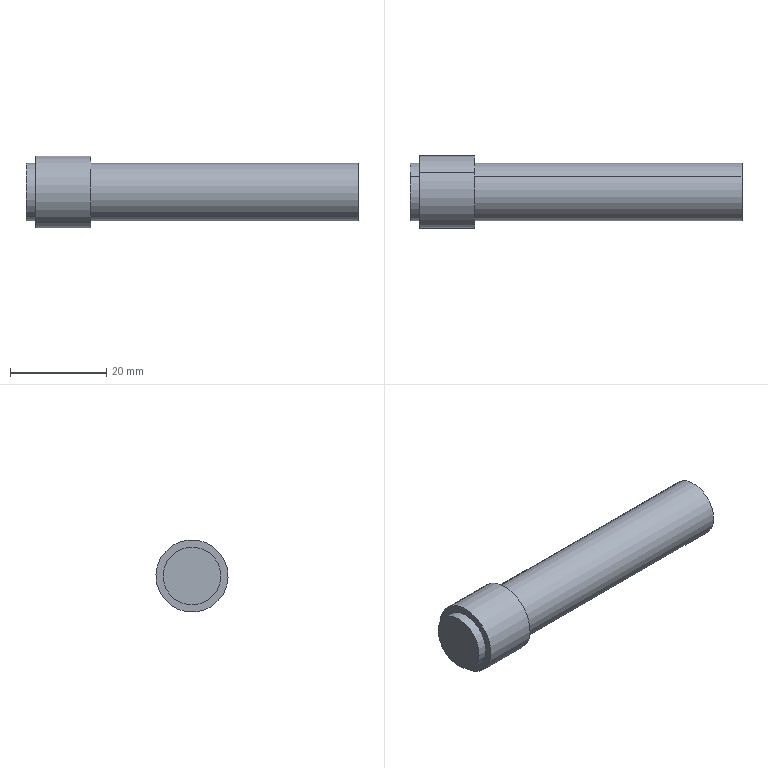Component | SolidWorks | GearShaft-4 | 1 solid | 10 faces | box 69 x 15 x 15 mm | volume 8535 mm3 | cylinder 6 | plane 4 | commonest cylinder face diameters 12 x4 15 x2
build123d program:
from build123d import *

# Parameters (mm, degrees)
BOSS_EXTRUDE1_DEPTH      = 14
BOSS_EXTRUDE1_DEPTH_BACK = 55
SKETCH1_R                = 6
BOSS_EXTRUDE2_START      = -2
SKETCH2_R                = 7.5
BOSS_EXTRUDE2_DEPTH      = 11.5


with BuildPart() as part:
    # Sketch1 → Boss-Extrude1 (new, two sides: drawn at the far end of the back side and taken through both)
    with BuildSketch(Plane.XY.offset(-BOSS_EXTRUDE1_DEPTH_BACK)):
        with Locations((-64.2, 0)):
            Circle(SKETCH1_R)
    extrude(amount=BOSS_EXTRUDE1_DEPTH + BOSS_EXTRUDE1_DEPTH_BACK)

    # Sketch2 → Boss-Extrude2 (add)
    with BuildSketch(Plane.XY.offset(14).offset(BOSS_EXTRUDE2_START)):
        with Locations((-64.2, 0)):
            Circle(SKETCH2_R)
    extrude(amount=-BOSS_EXTRUDE2_DEPTH)


solid = part.part

# Placed as in the assembly
solid = solid.moved(Location((-42.875, -67.172, 107.182), (0, -90, 0)))
STEP:
#1=COLOUR_RGB('',0.7922,0.8196,0.9333);
#2=FILL_AREA_STYLE_COLOUR('',#1);
#3=FILL_AREA_STYLE('',(#2));
#4=SURFACE_STYLE_FILL_AREA(#3);
#5=SURFACE_SIDE_STYLE('',(#4));
#6=SURFACE_STYLE_USAGE(.BOTH.,#5);
#7=PRESENTATION_STYLE_ASSIGNMENT((#6));
#8=CARTESIAN_POINT('',(-2.16,-2.518,1.892));
#9=VERTEX_POINT('',#8);
#10=CARTESIAN_POINT('',(-2.16,-2.771,1.493));
#11=VERTEX_POINT('',#10);
#12=CARTESIAN_POINT('',(-2.16,-2.645,1.692));
#13=DIRECTION('',(1.,0.,0.));
#14=DIRECTION('',(0.,-0.5345,-0.8452));
#15=AXIS2_PLACEMENT_3D('',#12,#13,#14);
#16=CIRCLE('',#15,0.2362);
#17=EDGE_CURVE('',#9,#11,#16,.T.);
#18=ORIENTED_EDGE('',*,*,#17,.F.);
#19=CARTESIAN_POINT('',(-2.239,-2.518,1.892));
#20=VERTEX_POINT('',#19);
#21=CARTESIAN_POINT('',(0.4773,-2.518,1.892));
#22=DIRECTION('',(-1.,-0.,-0.));
#23=VECTOR('',#22,39.37);
#24=LINE('',#21,#23);
#25=EDGE_CURVE('',#9,#20,#24,.T.);
#26=ORIENTED_EDGE('',*,*,#25,.T.);
#27=CARTESIAN_POINT('',(-2.239,-2.771,1.493));
#28=VERTEX_POINT('',#27);
#29=CARTESIAN_POINT('',(-2.239,-2.645,1.692));
#30=DIRECTION('',(-1.,-0.,-0.));
#31=DIRECTION('',(0.,-0.5345,-0.8452));
#32=AXIS2_PLACEMENT_3D('',#29,#30,#31);
#33=CIRCLE('',#32,0.2362);
#34=EDGE_CURVE('',#28,#20,#33,.T.);
#35=ORIENTED_EDGE('',*,*,#34,.F.);
#36=CARTESIAN_POINT('',(0.4773,-2.771,1.493));
#37=DIRECTION('',(-1.,-0.,-0.));
#38=VECTOR('',#37,39.37);
#39=LINE('',#36,#38);
#40=EDGE_CURVE('',#11,#28,#39,.T.);
#41=ORIENTED_EDGE('',*,*,#40,.F.);
#42=EDGE_LOOP('',(#18,#26,#35,#41));
#43=FACE_OUTER_BOUND('',#42,.T.);
#44=CARTESIAN_POINT('',(0.4773,-2.645,1.692));
#45=DIRECTION('',(-1.,-0.,-0.));
#46=DIRECTION('',(0.,-0.5345,-0.8452));
#47=AXIS2_PLACEMENT_3D('',#44,#45,#46);
#48=CYLINDRICAL_SURFACE('',#47,0.2362);
#49=ADVANCED_FACE('',(#43),#48,.T.);
#50=CARTESIAN_POINT('',(-1.708,-2.802,1.443));
#51=VERTEX_POINT('',#50);
#52=CARTESIAN_POINT('',(-1.708,-2.487,1.942));
#53=VERTEX_POINT('',#52);
#54=CARTESIAN_POINT('',(-1.708,-2.645,1.692));
#55=DIRECTION('',(-1.,-0.,-0.));
#56=DIRECTION('',(0.,-0.5345,-0.8452));
#57=AXIS2_PLACEMENT_3D('',#54,#55,#56);
#58=CIRCLE('',#57,0.2953);
#59=EDGE_CURVE('',#51,#53,#58,.T.);
#60=ORIENTED_EDGE('',*,*,#59,.T.);
#61=CARTESIAN_POINT('',(-2.16,-2.487,1.942));
#62=VERTEX_POINT('',#61);
#63=CARTESIAN_POINT('',(-1.708,-2.487,1.942));
#64=DIRECTION('',(-1.,-0.,-0.));
#65=VECTOR('',#64,39.37);
#66=LINE('',#63,#65);
#67=EDGE_CURVE('',#53,#62,#66,.T.);
#68=ORIENTED_EDGE('',*,*,#67,.T.);
#69=CARTESIAN_POINT('',(-2.16,-2.802,1.443));
#70=VERTEX_POINT('',#69);
#71=CARTESIAN_POINT('',(-2.16,-2.645,1.692));
#72=DIRECTION('',(-1.,-0.,-0.));
#73=DIRECTION('',(0.,-0.5345,-0.8452));
#74=AXIS2_PLACEMENT_3D('',#71,#72,#73);
#75=CIRCLE('',#74,0.2953);
#76=EDGE_CURVE('',#70,#62,#75,.T.);
#77=ORIENTED_EDGE('',*,*,#76,.F.);
#78=CARTESIAN_POINT('',(-1.708,-2.802,1.443));
#79=DIRECTION('',(-1.,-0.,-0.));
#80=VECTOR('',#79,39.37);
#81=LINE('',#78,#80);
#82=EDGE_CURVE('',#51,#70,#81,.T.);
#83=ORIENTED_EDGE('',*,*,#82,.F.);
#84=EDGE_LOOP('',(#60,#68,#77,#83));
#85=FACE_OUTER_BOUND('',#84,.T.);
#86=CARTESIAN_POINT('',(-1.708,-2.645,1.692));
#87=DIRECTION('',(-1.,-0.,-0.));
#88=DIRECTION('',(0.,-0.5345,-0.8452));
#89=AXIS2_PLACEMENT_3D('',#86,#87,#88);
#90=CYLINDRICAL_SURFACE('',#89,0.2953);
#91=ADVANCED_FACE('',(#85),#90,.T.);
#92=CARTESIAN_POINT('',(0.4773,-2.771,1.493));
#93=VERTEX_POINT('',#92);
#94=CARTESIAN_POINT('',(0.4773,-2.518,1.892));
#95=VERTEX_POINT('',#94);
#96=CARTESIAN_POINT('',(0.4773,-2.645,1.692));
#97=DIRECTION('',(-1.,-0.,-0.));
#98=DIRECTION('',(0.,-0.5345,-0.8452));
#99=AXIS2_PLACEMENT_3D('',#96,#97,#98);
#100=CIRCLE('',#99,0.2362);
#101=EDGE_CURVE('',#93,#95,#100,.T.);
#102=ORIENTED_EDGE('',*,*,#101,.T.);
#103=CARTESIAN_POINT('',(-1.708,-2.518,1.892));
#104=VERTEX_POINT('',#103);
#105=CARTESIAN_POINT('',(0.4773,-2.518,1.892));
#106=DIRECTION('',(-1.,-0.,-0.));
#107=VECTOR('',#106,39.37);
#108=LINE('',#105,#107);
#109=EDGE_CURVE('',#95,#104,#108,.T.);
#110=ORIENTED_EDGE('',*,*,#109,.T.);
#111=CARTESIAN_POINT('',(-1.708,-2.771,1.493));
#112=VERTEX_POINT('',#111);
#113=CARTESIAN_POINT('',(-1.708,-2.645,1.692));
#114=DIRECTION('',(1.,0.,0.));
#115=DIRECTION('',(0.,-0.5345,-0.8452));
#116=AXIS2_PLACEMENT_3D('',#113,#114,#115);
#117=CIRCLE('',#116,0.2362);
#118=EDGE_CURVE('',#104,#112,#117,.T.);
#119=ORIENTED_EDGE('',*,*,#118,.T.);
#120=CARTESIAN_POINT('',(0.4773,-2.771,1.493));
#121=DIRECTION('',(-1.,-0.,-0.));
#122=VECTOR('',#121,39.37);
#123=LINE('',#120,#122);
#124=EDGE_CURVE('',#93,#112,#123,.T.);
#125=ORIENTED_EDGE('',*,*,#124,.F.);
#126=EDGE_LOOP('',(#102,#110,#119,#125));
#127=FACE_OUTER_BOUND('',#126,.T.);
#128=CARTESIAN_POINT('',(0.4773,-2.645,1.692));
#129=DIRECTION('',(-1.,-0.,-0.));
#130=DIRECTION('',(0.,-0.5345,-0.8452));
#131=AXIS2_PLACEMENT_3D('',#128,#129,#130);
#132=CYLINDRICAL_SURFACE('',#131,0.2362);
#133=ADVANCED_FACE('',(#127),#132,.T.);
#134=ORIENTED_EDGE('',*,*,#109,.F.);
#135=CARTESIAN_POINT('',(0.4773,-2.645,1.692));
#136=DIRECTION('',(-1.,-0.,-0.));
#137=DIRECTION('',(0.,-0.5345,-0.8452));
#138=AXIS2_PLACEMENT_3D('',#135,#136,#137);
#139=CIRCLE('',#138,0.2362);
#140=EDGE_CURVE('',#95,#93,#139,.T.);
#141=ORIENTED_EDGE('',*,*,#140,.T.);
#142=ORIENTED_EDGE('',*,*,#124,.T.);
#143=CARTESIAN_POINT('',(-1.708,-2.645,1.692));
#144=DIRECTION('',(1.,0.,0.));
#145=DIRECTION('',(0.,-0.5345,-0.8452));
#146=AXIS2_PLACEMENT_3D('',#143,#144,#145);
#147=CIRCLE('',#146,0.2362);
#148=EDGE_CURVE('',#112,#104,#147,.T.);
#149=ORIENTED_EDGE('',*,*,#148,.T.);
#150=EDGE_LOOP('',(#134,#141,#142,#149));
#151=FACE_OUTER_BOUND('',#150,.T.);
#152=CARTESIAN_POINT('',(0.4773,-2.645,1.692));
#153=DIRECTION('',(-1.,-0.,-0.));
#154=DIRECTION('',(0.,-0.5345,-0.8452));
#155=AXIS2_PLACEMENT_3D('',#152,#153,#154);
#156=CYLINDRICAL_SURFACE('',#155,0.2362);
#157=ADVANCED_FACE('',(#151),#156,.T.);
#158=ORIENTED_EDGE('',*,*,#101,.F.);
#159=ORIENTED_EDGE('',*,*,#140,.F.);
#160=EDGE_LOOP('',(#158,#159));
#161=FACE_OUTER_BOUND('',#160,.T.);
#162=CARTESIAN_POINT('',(0.4773,-2.645,1.692));
#163=DIRECTION('',(-1.,-0.,-0.));
#164=DIRECTION('',(0.,-0.5345,-0.8452));
#165=AXIS2_PLACEMENT_3D('',#162,#163,#164);
#166=PLANE('',#165);
#167=ADVANCED_FACE('',(#161),#166,.F.);
#168=ORIENTED_EDGE('',*,*,#67,.F.);
#169=CARTESIAN_POINT('',(-1.708,-2.645,1.692));
#170=DIRECTION('',(-1.,-0.,-0.));
#171=DIRECTION('',(0.,-0.5345,-0.8452));
#172=AXIS2_PLACEMENT_3D('',#169,#170,#171);
#173=CIRCLE('',#172,0.2953);
#174=EDGE_CURVE('',#53,#51,#173,.T.);
#175=ORIENTED_EDGE('',*,*,#174,.T.);
#176=ORIENTED_EDGE('',*,*,#82,.T.);
#177=CARTESIAN_POINT('',(-2.16,-2.645,1.692));
#178=DIRECTION('',(-1.,-0.,-0.));
#179=DIRECTION('',(0.,-0.5345,-0.8452));
#180=AXIS2_PLACEMENT_3D('',#177,#178,#179);
#181=CIRCLE('',#180,0.2953);
#182=EDGE_CURVE('',#62,#70,#181,.T.);
#183=ORIENTED_EDGE('',*,*,#182,.F.);
#184=EDGE_LOOP('',(#168,#175,#176,#183));
#185=FACE_OUTER_BOUND('',#184,.T.);
#186=CARTESIAN_POINT('',(-1.708,-2.645,1.692));
#187=DIRECTION('',(-1.,-0.,-0.));
#188=DIRECTION('',(0.,-0.5345,-0.8452));
#189=AXIS2_PLACEMENT_3D('',#186,#187,#188);
#190=CYLINDRICAL_SURFACE('',#189,0.2953);
#191=ADVANCED_FACE('',(#185),#190,.T.);
#192=ORIENTED_EDGE('',*,*,#148,.F.);
#193=ORIENTED_EDGE('',*,*,#118,.F.);
#194=EDGE_LOOP('',(#192,#193));
#195=FACE_BOUND('',#194,.T.);
#196=ORIENTED_EDGE('',*,*,#59,.F.);
#197=ORIENTED_EDGE('',*,*,#174,.F.);
#198=EDGE_LOOP('',(#196,#197));
#199=FACE_OUTER_BOUND('',#198,.T.);
#200=CARTESIAN_POINT('',(-1.708,-2.645,1.692));
#201=DIRECTION('',(-1.,-0.,-0.));
#202=DIRECTION('',(0.,-0.5345,-0.8452));
#203=AXIS2_PLACEMENT_3D('',#200,#201,#202);
#204=PLANE('',#203);
#205=ADVANCED_FACE('',(#195,#199),#204,.F.);
#206=CARTESIAN_POINT('',(-2.16,-2.645,1.692));
#207=DIRECTION('',(1.,0.,0.));
#208=DIRECTION('',(0.,-0.5345,-0.8452));
#209=AXIS2_PLACEMENT_3D('',#206,#207,#208);
#210=CIRCLE('',#209,0.2362);
#211=EDGE_CURVE('',#11,#9,#210,.T.);
#212=ORIENTED_EDGE('',*,*,#211,.T.);
#213=ORIENTED_EDGE('',*,*,#17,.T.);
#214=EDGE_LOOP('',(#212,#213));
#215=FACE_BOUND('',#214,.T.);
#216=ORIENTED_EDGE('',*,*,#76,.T.);
#217=ORIENTED_EDGE('',*,*,#182,.T.);
#218=EDGE_LOOP('',(#216,#217));
#219=FACE_OUTER_BOUND('',#218,.T.);
#220=CARTESIAN_POINT('',(-2.16,-2.645,1.692));
#221=DIRECTION('',(-1.,-0.,-0.));
#222=DIRECTION('',(0.,-0.5345,-0.8452));
#223=AXIS2_PLACEMENT_3D('',#220,#221,#222);
#224=PLANE('',#223);
#225=ADVANCED_FACE('',(#215,#219),#224,.T.);
#226=ORIENTED_EDGE('',*,*,#34,.T.);
#227=CARTESIAN_POINT('',(-2.239,-2.645,1.692));
#228=DIRECTION('',(-1.,-0.,-0.));
#229=DIRECTION('',(0.,-0.5345,-0.8452));
#230=AXIS2_PLACEMENT_3D('',#227,#228,#229);
#231=CIRCLE('',#230,0.2362);
#232=EDGE_CURVE('',#20,#28,#231,.T.);
#233=ORIENTED_EDGE('',*,*,#232,.T.);
#234=EDGE_LOOP('',(#226,#233));
#235=FACE_OUTER_BOUND('',#234,.T.);
#236=CARTESIAN_POINT('',(-2.239,-2.645,1.692));
#237=DIRECTION('',(-1.,-0.,-0.));
#238=DIRECTION('',(0.,-0.5345,-0.8452));
#239=AXIS2_PLACEMENT_3D('',#236,#237,#238);
#240=PLANE('',#239);
#241=ADVANCED_FACE('',(#235),#240,.T.);
#242=ORIENTED_EDGE('',*,*,#25,.F.);
#243=ORIENTED_EDGE('',*,*,#211,.F.);
#244=ORIENTED_EDGE('',*,*,#40,.T.);
#245=ORIENTED_EDGE('',*,*,#232,.F.);
#246=EDGE_LOOP('',(#242,#243,#244,#245));
#247=FACE_OUTER_BOUND('',#246,.T.);
#248=CARTESIAN_POINT('',(0.4773,-2.645,1.692));
#249=DIRECTION('',(-1.,-0.,-0.));
#250=DIRECTION('',(0.,-0.5345,-0.8452));
#251=AXIS2_PLACEMENT_3D('',#248,#249,#250);
#252=CYLINDRICAL_SURFACE('',#251,0.2362);
#253=ADVANCED_FACE('',(#247),#252,.T.);
#254=CLOSED_SHELL('',(#49,#91,#133,#157,#167,#191,#205,#225,#241,#253));
#255=MANIFOLD_SOLID_BREP('',#254);
#256=STYLED_ITEM('',(#7),#255);
#257=(LENGTH_UNIT()NAMED_UNIT(*)SI_UNIT($,.METRE.));
#258=LENGTH_MEASURE_WITH_UNIT(LENGTH_MEASURE(0.0254),#257);
#259=DIMENSIONAL_EXPONENTS(1.,0.,0.,0.,0.,0.,0.);
#260=(CONVERSION_BASED_UNIT('',#258)LENGTH_UNIT()NAMED_UNIT(#259));
#261=UNCERTAINTY_MEASURE_WITH_UNIT(LENGTH_MEASURE(0.00001),#260,'','');
#262=(NAMED_UNIT(*)PLANE_ANGLE_UNIT()SI_UNIT($,.RADIAN.));
#263=(NAMED_UNIT(*)SI_UNIT($,.STERADIAN.)SOLID_ANGLE_UNIT());
#264=(GEOMETRIC_REPRESENTATION_CONTEXT(3)GLOBAL_UNCERTAINTY_ASSIGNED_CONTEXT((#261))GLOBAL_UNIT_ASSIGNED_CONTEXT((#260,#262,#263))REPRESENTATION_CONTEXT('',''));
#265=MECHANICAL_DESIGN_GEOMETRIC_PRESENTATION_REPRESENTATION('',(#256),#264);
#266=PRESENTATION_LAYER_ASSIGNMENT('','',(#256));
#267=CARTESIAN_POINT('',(0.,0.,0.));
#268=DIRECTION('',(0.,0.,1.));
#269=DIRECTION('',(1.,0.,0.));
#270=AXIS2_PLACEMENT_3D('',#267,#268,#269);
#271=(LENGTH_UNIT()NAMED_UNIT(*)SI_UNIT($,.METRE.));
#272=LENGTH_MEASURE_WITH_UNIT(LENGTH_MEASURE(0.0254),#271);
#273=DIMENSIONAL_EXPONENTS(1.,0.,0.,0.,0.,0.,0.);
#274=(CONVERSION_BASED_UNIT('',#272)LENGTH_UNIT()NAMED_UNIT(#273));
#275=UNCERTAINTY_MEASURE_WITH_UNIT(LENGTH_MEASURE(0.00001),#274,'','');
#276=(NAMED_UNIT(*)PLANE_ANGLE_UNIT()SI_UNIT($,.RADIAN.));
#277=(NAMED_UNIT(*)SI_UNIT($,.STERADIAN.)SOLID_ANGLE_UNIT());
#278=(GEOMETRIC_REPRESENTATION_CONTEXT(3)GLOBAL_UNCERTAINTY_ASSIGNED_CONTEXT((#275))GLOBAL_UNIT_ASSIGNED_CONTEXT((#274,#276,#277))REPRESENTATION_CONTEXT('',''));
#279=ADVANCED_BREP_SHAPE_REPRESENTATION('',(#255,#270),#278);